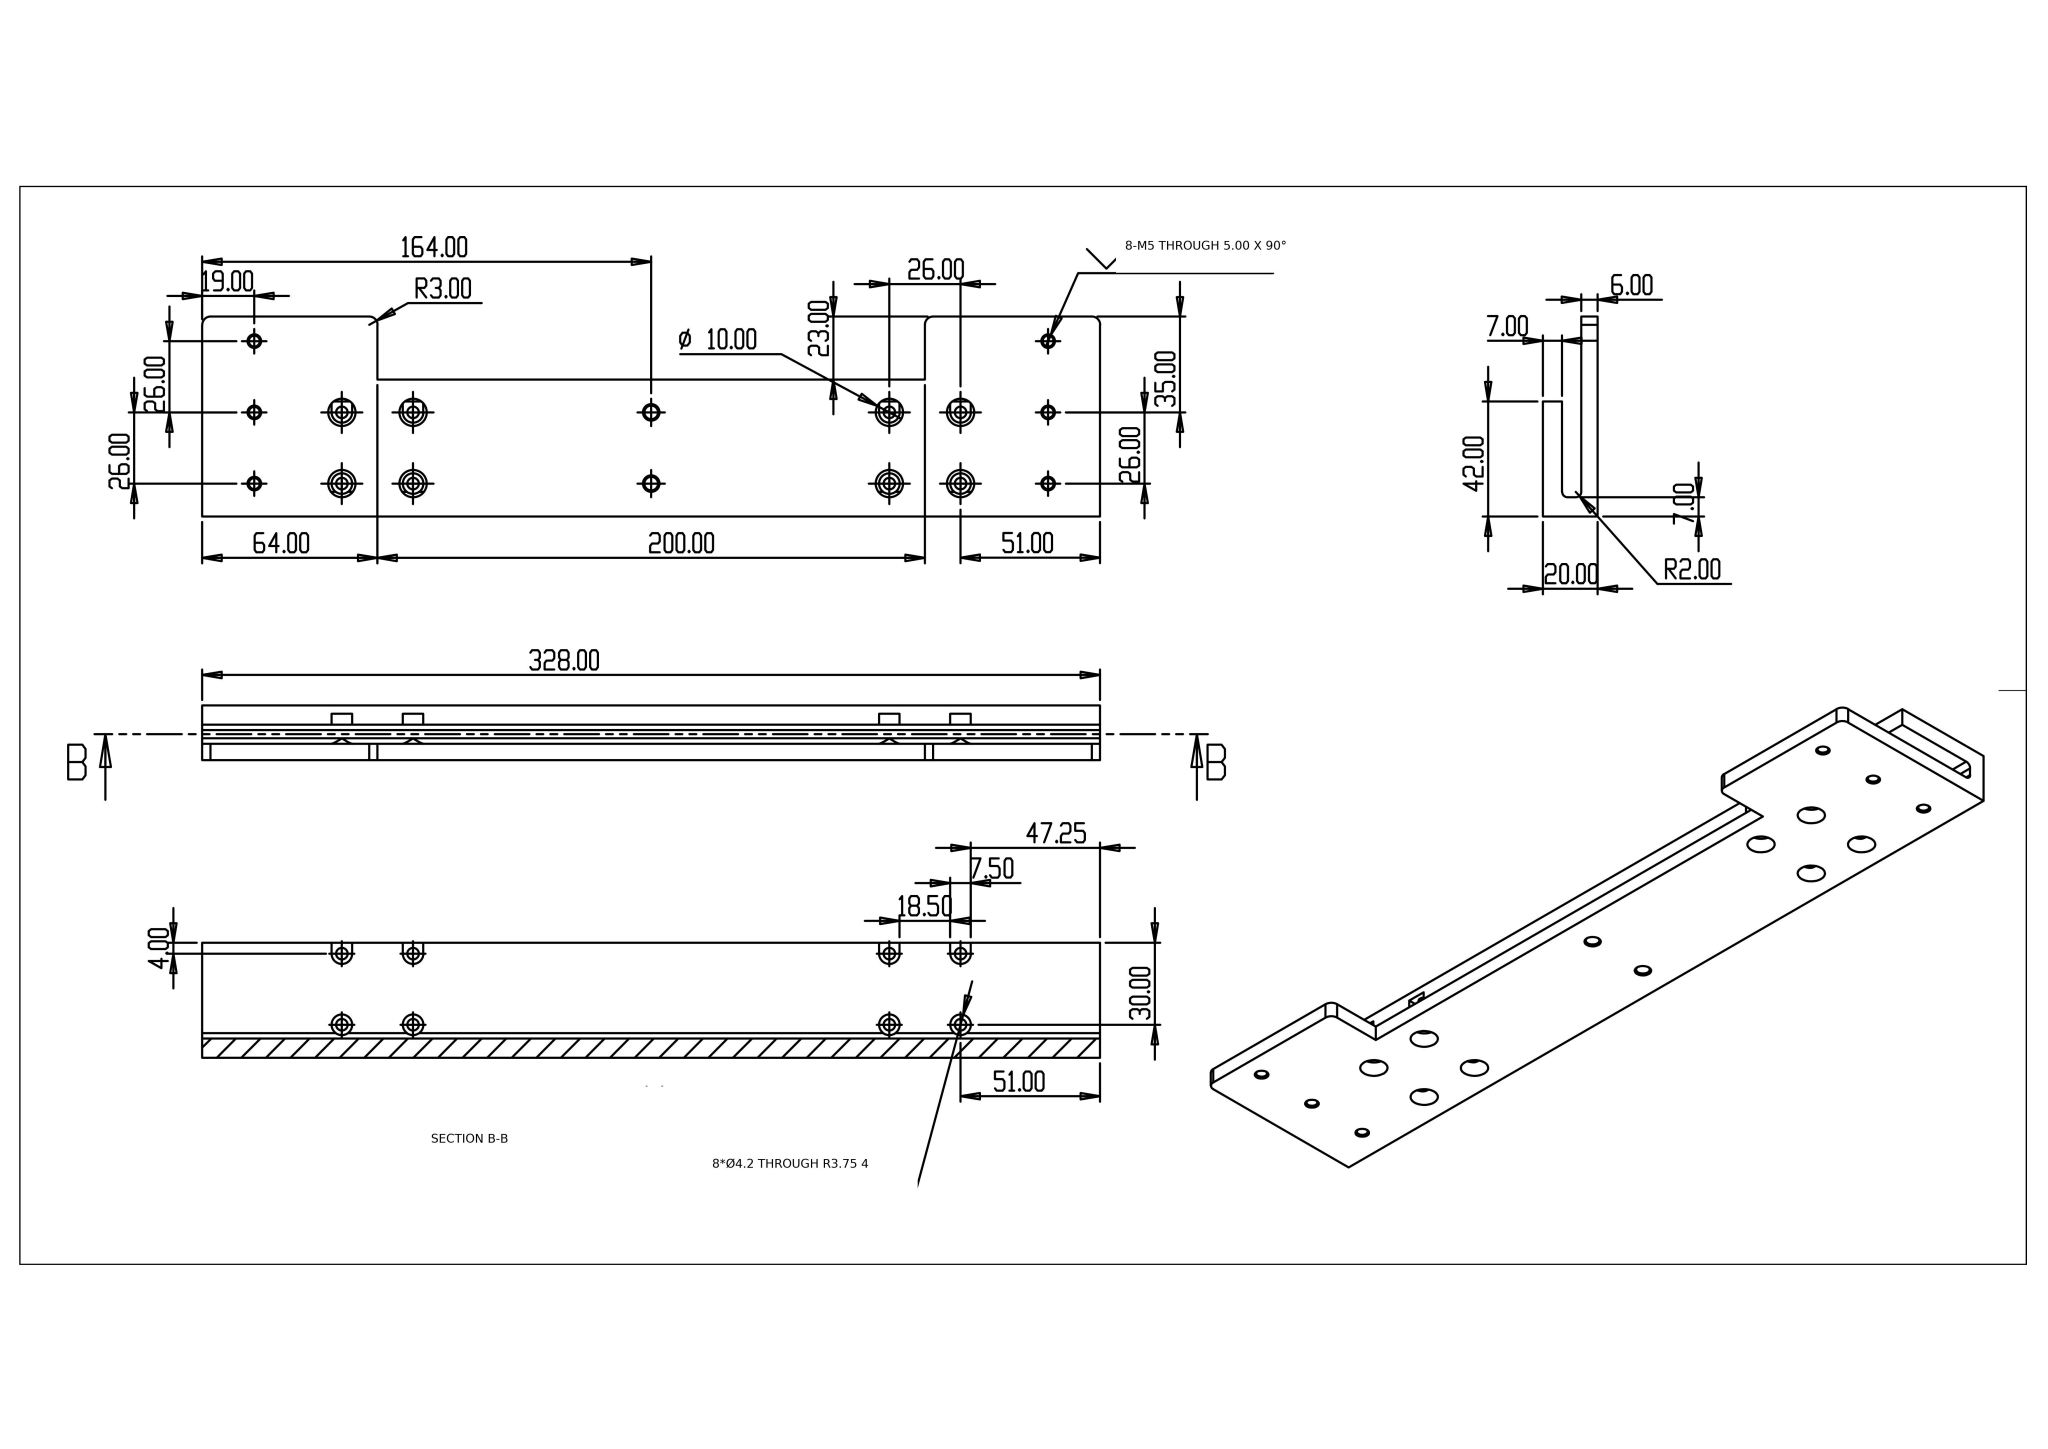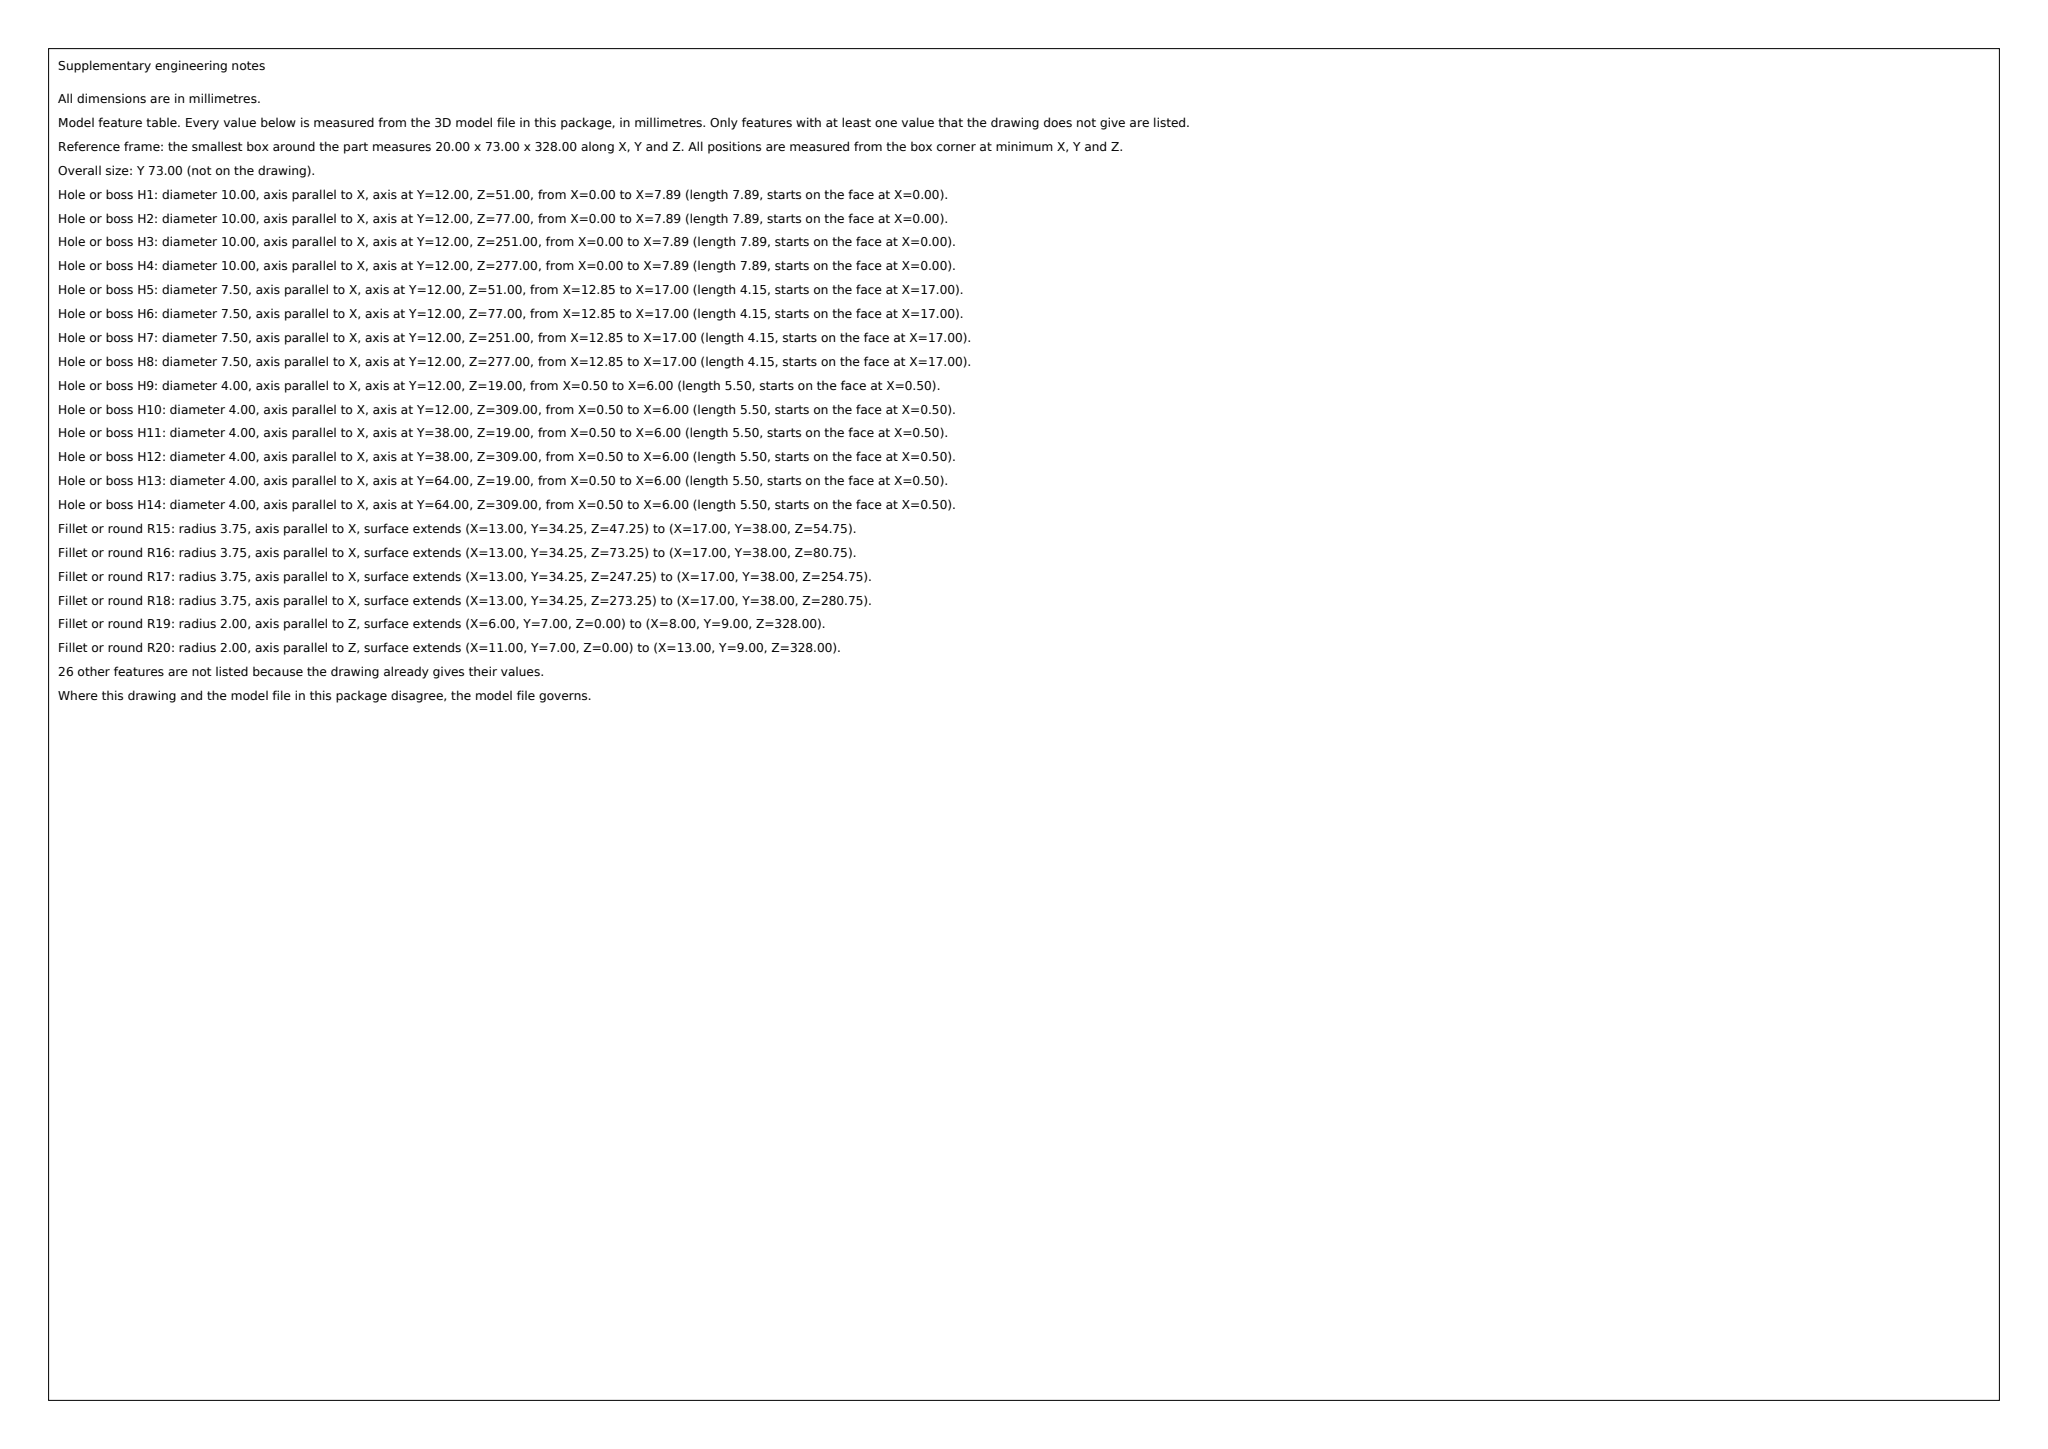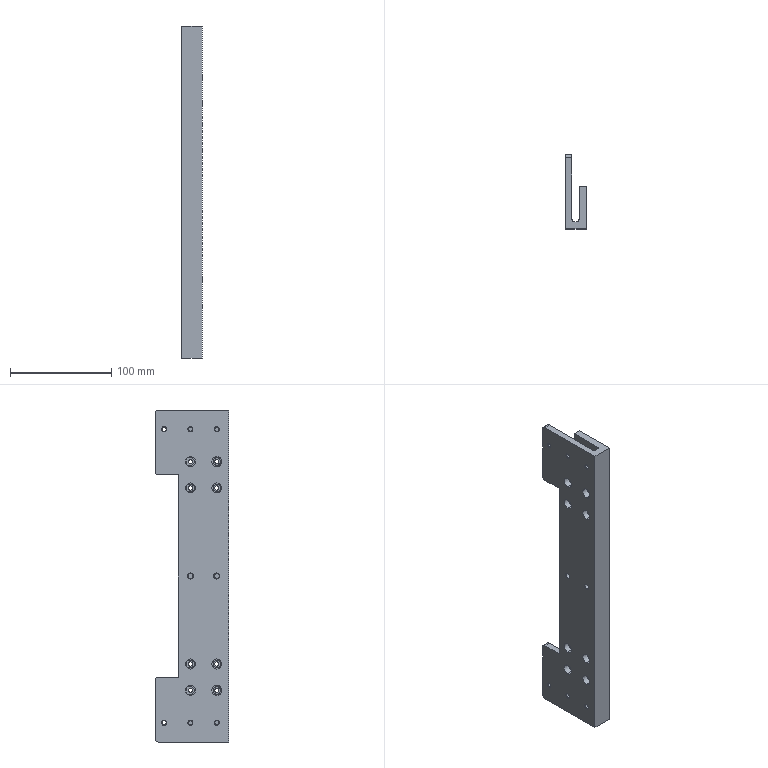Part | SolidWorks | mm | 1 solid | 112 faces | box 20 x 73 x 328 mm | volume 222727 mm3 | cylinder 66 | plane 30 | cone 16 | commonest cylinder face diameters 10 x16 4.2 x16 4 x14 7.5 x12 5 x4 6 x4
build123d program:
from build123d import *

# Parameters (mm, degrees)
BOSS_EXTRUDE1_DEPTH            = 328
CUT_EXTRUDE1_DEPTH             = 332.282
CUT_EXTRUDE2_REACH             = 333.282
SKETCH3_R                      = 2
CHAMFER1_SIZE                  = 0.5
SKETCH4_R                      = 3.75
SKETCH4_R_2                    = 3.75
CUT_EXTRUDE3_DEPTH             = 4
CUT_EXTRUDE3_DIRECTION_2_REACH = 332.934


with BuildPart() as part:
    # Sketch1 → Boss-Extrude1 (new body)
    with BuildSketch(Plane.XY):
        with BuildLine():
            Line((-20, 28), (-20, -42))
            Line((-20, -42), (0, -42))
            Line((0, -42), (0, 0))
            Line((0, 0), (-7, 0))
            Line((-7, 0), (-7, -33))
            ThreePointArc((-7, -33), (-7.586, -34.414), (-9, -35))
            Line((-9, -35), (-12, -35))
            ThreePointArc((-12, -35), (-13.414, -34.414), (-14, -33))
            Line((-14, -33), (-14, 28))
            Line((-14, 28), (-14, 31))
            Line((-14, 31), (-20, 31))
            Line((-20, 31), (-20, 28))
        make_face()
    extrude(amount=BOSS_EXTRUDE1_DEPTH)

    # Sketch2 → Cut-Extrude1 (cut, through all)
    with BuildSketch(Plane(origin=(0, 0, 0), x_dir=(0, 0, -1), z_dir=(1, 0, 0))):
        with BuildLine():
            Line((-64, 28), (-64, 8))
            Line((-64, 8), (-264, 8))
            Line((-264, 8), (-264, 28))
            ThreePointArc((-264, 28), (-264.879, 30.121), (-267, 31))
            Line((-267, 31), (-61, 31))
            ThreePointArc((-61, 31), (-63.121, 30.121), (-64, 28))
        make_face()
        with BuildLine():
            Line((-328, 28), (-328, 31))
            Line((-328, 31), (-325, 31))
            ThreePointArc((-325, 31), (-327.121, 30.121), (-328, 28))
        make_face()
        with BuildLine():
            Line((-3, 31), (0, 31))
            Line((0, 31), (0, 28))
            ThreePointArc((0, 28), (-0.8787, 30.121), (-3, 31))
        make_face()
        with BuildLine():
            ThreePointArc((-307, 22), (-309, 24), (-311, 22))
            ThreePointArc((-311, 22), (-309, 20), (-307, 22))
        make_face()
        with BuildLine():
            ThreePointArc((-17, 22), (-19, 24), (-21, 22))
            ThreePointArc((-21, 22), (-19, 20), (-17, 22))
        make_face()
        with BuildLine():
            ThreePointArc((-53.1, -4), (-51, -6.1), (-48.9, -4))
            ThreePointArc((-48.9, -4), (-51, -1.9), (-53.1, -4))
        make_face()
        with BuildLine():
            ThreePointArc((-253.1, -30), (-251, -32.1), (-248.9, -30))
            ThreePointArc((-248.9, -30), (-251, -27.9), (-253.1, -30))
        make_face()
        with BuildLine():
            ThreePointArc((-279.1, -30), (-277, -32.1), (-274.9, -30))
            ThreePointArc((-274.9, -30), (-277, -27.9), (-279.1, -30))
        make_face()
        with BuildLine():
            ThreePointArc((-253.1, -4), (-251, -6.1), (-248.9, -4))
            ThreePointArc((-248.9, -4), (-251, -1.9), (-253.1, -4))
        make_face()
        with BuildLine():
            ThreePointArc((-279.1, -4), (-277, -6.1), (-274.9, -4))
            ThreePointArc((-274.9, -4), (-277, -1.9), (-279.1, -4))
        make_face()
        with BuildLine():
            ThreePointArc((-79.1, -30), (-77, -32.1), (-74.9, -30))
            ThreePointArc((-74.9, -30), (-77, -27.9), (-79.1, -30))
        make_face()
        with BuildLine():
            ThreePointArc((-53.1, -30), (-51, -32.1), (-48.9, -30))
            ThreePointArc((-48.9, -30), (-51, -27.9), (-53.1, -30))
        make_face()
        with BuildLine():
            ThreePointArc((-79.1, -4), (-77, -6.1), (-74.9, -4))
            ThreePointArc((-74.9, -4), (-77, -1.9), (-79.1, -4))
        make_face()
    extrude(amount=-CUT_EXTRUDE1_DEPTH, mode=Mode.SUBTRACT)

    # Sketch3 → Cut-Extrude2 (cut, up to next)
    with BuildSketch(Plane.ZY.offset(20), mode=Mode.PRIVATE) as cut_extrude2_sk1:
        with Locations((309, -3.997)):
            Circle(SKETCH3_R)
    cut_extrude2_tool1 = extrude(cut_extrude2_sk1.sketch, amount=-CUT_EXTRUDE2_REACH, mode=Mode.PRIVATE) & part.part
    # Sketch3 → Cut-Extrude2 (cut, up to next)
    with BuildSketch(Plane.ZY.offset(20), mode=Mode.PRIVATE) as cut_extrude2_sk2:
        with Locations((309, -29.997)):
            Circle(SKETCH3_R)
    cut_extrude2_tool2 = extrude(cut_extrude2_sk2.sketch, amount=-CUT_EXTRUDE2_REACH, mode=Mode.PRIVATE) & part.part
    # Sketch3 → Cut-Extrude2 (cut, up to next)
    with BuildSketch(Plane.ZY.offset(20), mode=Mode.PRIVATE) as cut_extrude2_sk3:
        with Locations((19, -3.997)):
            Circle(SKETCH3_R)
    cut_extrude2_tool3 = extrude(cut_extrude2_sk3.sketch, amount=-CUT_EXTRUDE2_REACH, mode=Mode.PRIVATE) & part.part
    # Sketch3 → Cut-Extrude2 (cut, up to next)
    with BuildSketch(Plane.ZY.offset(20), mode=Mode.PRIVATE) as cut_extrude2_sk4:
        with Locations((19, -29.997)):
            Circle(SKETCH3_R)
    cut_extrude2_tool4 = extrude(cut_extrude2_sk4.sketch, amount=-CUT_EXTRUDE2_REACH, mode=Mode.PRIVATE) & part.part
    # Sketch3 → Cut-Extrude2 (cut, up to next)
    with BuildSketch(Plane.ZY.offset(20), mode=Mode.PRIVATE) as cut_extrude2_sk5:
        with BuildLine():
            ThreePointArc((282, -29.997), (277, -24.997), (272, -29.997))
            ThreePointArc((272, -29.997), (277, -34.997), (282, -29.997))
        make_face()
    cut_extrude2_tool5 = extrude(cut_extrude2_sk5.sketch, amount=-CUT_EXTRUDE2_REACH, mode=Mode.PRIVATE) & part.part
    # Sketch3 → Cut-Extrude2 (cut, up to next)
    with BuildSketch(Plane.ZY.offset(20), mode=Mode.PRIVATE) as cut_extrude2_sk6:
        with BuildLine():
            ThreePointArc((164, -27.497), (161.5, -29.997), (164, -32.497))
            ThreePointArc((164, -32.497), (166.5, -29.997), (164, -27.497))
        make_face()
    cut_extrude2_tool6 = extrude(cut_extrude2_sk6.sketch, amount=-CUT_EXTRUDE2_REACH, mode=Mode.PRIVATE) & part.part
    # Sketch3 → Cut-Extrude2 (cut, up to next)
    with BuildSketch(Plane.ZY.offset(20), mode=Mode.PRIVATE) as cut_extrude2_sk7:
        with BuildLine():
            ThreePointArc((164, -1.497), (161.5, -3.997), (164, -6.497))
            ThreePointArc((164, -6.497), (166.5, -3.997), (164, -1.497))
        make_face()
    cut_extrude2_tool7 = extrude(cut_extrude2_sk7.sketch, amount=-CUT_EXTRUDE2_REACH, mode=Mode.PRIVATE) & part.part
    # Sketch3 → Cut-Extrude2 (cut, up to next)
    with BuildSketch(Plane.ZY.offset(20), mode=Mode.PRIVATE) as cut_extrude2_sk8:
        with BuildLine():
            ThreePointArc((56, -3.997), (51, 1.003), (46, -3.997))
            ThreePointArc((46, -3.997), (51, -8.997), (56, -3.997))
        make_face()
    cut_extrude2_tool8 = extrude(cut_extrude2_sk8.sketch, amount=-CUT_EXTRUDE2_REACH, mode=Mode.PRIVATE) & part.part
    # Sketch3 → Cut-Extrude2 (cut, up to next)
    with BuildSketch(Plane.ZY.offset(20), mode=Mode.PRIVATE) as cut_extrude2_sk9:
        with BuildLine():
            ThreePointArc((82, -29.997), (77, -24.997), (72, -29.997))
            ThreePointArc((72, -29.997), (77, -34.997), (82, -29.997))
        make_face()
    cut_extrude2_tool9 = extrude(cut_extrude2_sk9.sketch, amount=-CUT_EXTRUDE2_REACH, mode=Mode.PRIVATE) & part.part
    # Sketch3 → Cut-Extrude2 (cut, up to next)
    with BuildSketch(Plane.ZY.offset(20), mode=Mode.PRIVATE) as cut_extrude2_sk10:
        with BuildLine():
            ThreePointArc((256, -29.997), (251, -24.997), (246, -29.997))
            ThreePointArc((246, -29.997), (251, -34.997), (256, -29.997))
        make_face()
    cut_extrude2_tool10 = extrude(cut_extrude2_sk10.sketch, amount=-CUT_EXTRUDE2_REACH, mode=Mode.PRIVATE) & part.part
    # Sketch3 → Cut-Extrude2 (cut, up to next)
    with BuildSketch(Plane.ZY.offset(20), mode=Mode.PRIVATE) as cut_extrude2_sk11:
        with BuildLine():
            ThreePointArc((256, -3.997), (251, 1.003), (246, -3.997))
            ThreePointArc((246, -3.997), (251, -8.997), (256, -3.997))
        make_face()
    cut_extrude2_tool11 = extrude(cut_extrude2_sk11.sketch, amount=-CUT_EXTRUDE2_REACH, mode=Mode.PRIVATE) & part.part
    # Sketch3 → Cut-Extrude2 (cut, up to next)
    with BuildSketch(Plane.ZY.offset(20), mode=Mode.PRIVATE) as cut_extrude2_sk12:
        with BuildLine():
            ThreePointArc((82, -3.997), (77, 1.003), (72, -3.997))
            ThreePointArc((72, -3.997), (77, -8.997), (82, -3.997))
        make_face()
    cut_extrude2_tool12 = extrude(cut_extrude2_sk12.sketch, amount=-CUT_EXTRUDE2_REACH, mode=Mode.PRIVATE) & part.part
    # Sketch3 → Cut-Extrude2 (cut, up to next)
    with BuildSketch(Plane.ZY.offset(20), mode=Mode.PRIVATE) as cut_extrude2_sk13:
        with BuildLine():
            ThreePointArc((56, -29.997), (51, -24.997), (46, -29.997))
            ThreePointArc((46, -29.997), (51, -34.997), (56, -29.997))
        make_face()
    cut_extrude2_tool13 = extrude(cut_extrude2_sk13.sketch, amount=-CUT_EXTRUDE2_REACH, mode=Mode.PRIVATE) & part.part
    # Sketch3 → Cut-Extrude2 (cut, up to next)
    with BuildSketch(Plane.ZY.offset(20), mode=Mode.PRIVATE) as cut_extrude2_sk14:
        with BuildLine():
            ThreePointArc((282, -3.997), (277, 1.003), (272, -3.997))
            ThreePointArc((272, -3.997), (277, -8.997), (282, -3.997))
        make_face()
    cut_extrude2_tool14 = extrude(cut_extrude2_sk14.sketch, amount=-CUT_EXTRUDE2_REACH, mode=Mode.PRIVATE) & part.part
    add(cut_extrude2_tool1.solids().sort_by_distance((-20, -3.997, 309))[0], mode=Mode.SUBTRACT)
    add(cut_extrude2_tool2.solids().sort_by_distance((-20, -29.997, 309))[0], mode=Mode.SUBTRACT)
    add(cut_extrude2_tool3.solids().sort_by_distance((-20, -3.997, 19))[0], mode=Mode.SUBTRACT)
    add(cut_extrude2_tool4.solids().sort_by_distance((-20, -29.997, 19))[0], mode=Mode.SUBTRACT)
    add(cut_extrude2_tool5.solids().sort_by_distance((-20, -29.997, 277))[0], mode=Mode.SUBTRACT)
    add(cut_extrude2_tool6.solids().sort_by_distance((-20, -29.997, 164))[0], mode=Mode.SUBTRACT)
    add(cut_extrude2_tool7.solids().sort_by_distance((-20, -3.997, 164))[0], mode=Mode.SUBTRACT)
    add(cut_extrude2_tool8.solids().sort_by_distance((-20, -3.997, 51))[0], mode=Mode.SUBTRACT)
    add(cut_extrude2_tool9.solids().sort_by_distance((-20, -29.997, 77))[0], mode=Mode.SUBTRACT)
    add(cut_extrude2_tool10.solids().sort_by_distance((-20, -29.997, 251))[0], mode=Mode.SUBTRACT)
    add(cut_extrude2_tool11.solids().sort_by_distance((-20, -3.997, 251))[0], mode=Mode.SUBTRACT)
    add(cut_extrude2_tool12.solids().sort_by_distance((-20, -3.997, 77))[0], mode=Mode.SUBTRACT)
    add(cut_extrude2_tool13.solids().sort_by_distance((-20, -29.997, 51))[0], mode=Mode.SUBTRACT)
    add(cut_extrude2_tool14.solids().sort_by_distance((-20, -3.997, 277))[0], mode=Mode.SUBTRACT)

    # Chamfer1
    chamfer1_edges = [part.edges().sort_by_distance(p)[0] for p in [
        (-20, 22, 311),
        (-20, 22, 17),
        (-20, -6.497, 164),
        (-20, -32.497, 164),
        (-20, -29.997, 17),
        (-20, -3.997, 17),
        (-20, -29.997, 307),
        (-20, -3.997, 307),
    ]]
    chamfer(chamfer1_edges, length=CHAMFER1_SIZE)

    # Sketch4 → Cut-Extrude3 (cut)
    with BuildSketch(Plane.ZY.offset(7)):
        with Locations(Location((51, -30, 0), (0, 0, 233.13))):
            Circle(SKETCH4_R)
        with Locations(Location((77, -30, 0), (0, 0, 233.13))):
            Circle(SKETCH4_R)
        with Locations(Location((251, -30, 0), (0, 0, 233.13))):
            Circle(SKETCH4_R)
        with Locations(Location((277, -30, 0), (0, 0, 233.13))):
            Circle(SKETCH4_R_2)
        with BuildLine():
            Line((47.25, -4), (47.25, 0))
            Line((47.25, 0), (54.75, 0))
            Line((54.75, 0), (54.75, -4))
            ThreePointArc((54.75, -4), (51, -7.75), (47.25, -4))
        make_face()
        with BuildLine():
            Line((280.75, 0), (280.75, -4))
            ThreePointArc((280.75, -4), (277, -7.75), (273.25, -4))
            Line((273.25, -4), (273.25, 0))
            Line((273.25, 0), (280.75, 0))
        make_face()
        with BuildLine():
            Line((254.75, 0), (254.75, -4))
            ThreePointArc((254.75, -4), (251, -7.75), (247.25, -4))
            Line((247.25, -4), (247.25, 0))
            Line((247.25, 0), (254.75, 0))
        make_face()
        with BuildLine():
            Line((80.75, 0), (80.75, -4))
            ThreePointArc((80.75, -4), (77, -7.75), (73.25, -4))
            Line((73.25, -4), (73.25, 0))
            Line((73.25, 0), (80.75, 0))
        make_face()
    extrude(amount=-CUT_EXTRUDE3_DEPTH, mode=Mode.SUBTRACT)

    # Cut-Extrude3 direction 2: up to this face of the body (flat: up to its plane)
    cut_extrude3_direction_2_end = Plane(part.part.faces().sort_by_distance((-14, -2.5, 3.342))[0])
    # Sketch4 → Cut-Extrude3 direction 2 (cut, up to the picked face)
    with BuildSketch(Plane.ZY.offset(7), mode=Mode.PRIVATE) as cut_extrude3_direction_2_sk1:
        with Locations(Location((51, -30, 0), (0, 0, 233.13))):
            Circle(SKETCH4_R)
    cut_extrude3_direction_2_tool1 = split(extrude(cut_extrude3_direction_2_sk1.sketch, amount=CUT_EXTRUDE3_DIRECTION_2_REACH, mode=Mode.PRIVATE), bisect_by=cut_extrude3_direction_2_end, keep=Keep.BOTH, mode=Mode.PRIVATE)
    # Sketch4 → Cut-Extrude3 direction 2 (cut, up to the picked face)
    with BuildSketch(Plane.ZY.offset(7), mode=Mode.PRIVATE) as cut_extrude3_direction_2_sk2:
        with Locations(Location((77, -30, 0), (0, 0, 233.13))):
            Circle(SKETCH4_R)
    cut_extrude3_direction_2_tool2 = split(extrude(cut_extrude3_direction_2_sk2.sketch, amount=CUT_EXTRUDE3_DIRECTION_2_REACH, mode=Mode.PRIVATE), bisect_by=cut_extrude3_direction_2_end, keep=Keep.BOTH, mode=Mode.PRIVATE)
    # Sketch4 → Cut-Extrude3 direction 2 (cut, up to the picked face)
    with BuildSketch(Plane.ZY.offset(7), mode=Mode.PRIVATE) as cut_extrude3_direction_2_sk3:
        with Locations(Location((251, -30, 0), (0, 0, 233.13))):
            Circle(SKETCH4_R)
    cut_extrude3_direction_2_tool3 = split(extrude(cut_extrude3_direction_2_sk3.sketch, amount=CUT_EXTRUDE3_DIRECTION_2_REACH, mode=Mode.PRIVATE), bisect_by=cut_extrude3_direction_2_end, keep=Keep.BOTH, mode=Mode.PRIVATE)
    # Sketch4 → Cut-Extrude3 direction 2 (cut, up to the picked face)
    with BuildSketch(Plane.ZY.offset(7), mode=Mode.PRIVATE) as cut_extrude3_direction_2_sk4:
        with Locations(Location((277, -30, 0), (0, 0, 233.13))):
            Circle(SKETCH4_R_2)
    cut_extrude3_direction_2_tool4 = split(extrude(cut_extrude3_direction_2_sk4.sketch, amount=CUT_EXTRUDE3_DIRECTION_2_REACH, mode=Mode.PRIVATE), bisect_by=cut_extrude3_direction_2_end, keep=Keep.BOTH, mode=Mode.PRIVATE)
    # Sketch4 → Cut-Extrude3 direction 2 (cut, up to the picked face)
    with BuildSketch(Plane.ZY.offset(7), mode=Mode.PRIVATE) as cut_extrude3_direction_2_sk5:
        with BuildLine():
            Line((47.25, -4), (47.25, 0))
            Line((47.25, 0), (54.75, 0))
            Line((54.75, 0), (54.75, -4))
            ThreePointArc((54.75, -4), (51, -7.75), (47.25, -4))
        make_face()
    cut_extrude3_direction_2_tool5 = split(extrude(cut_extrude3_direction_2_sk5.sketch, amount=CUT_EXTRUDE3_DIRECTION_2_REACH, mode=Mode.PRIVATE), bisect_by=cut_extrude3_direction_2_end, keep=Keep.BOTH, mode=Mode.PRIVATE)
    # Sketch4 → Cut-Extrude3 direction 2 (cut, up to the picked face)
    with BuildSketch(Plane.ZY.offset(7), mode=Mode.PRIVATE) as cut_extrude3_direction_2_sk6:
        with BuildLine():
            Line((280.75, 0), (280.75, -4))
            ThreePointArc((280.75, -4), (277, -7.75), (273.25, -4))
            Line((273.25, -4), (273.25, 0))
            Line((273.25, 0), (280.75, 0))
        make_face()
    cut_extrude3_direction_2_tool6 = split(extrude(cut_extrude3_direction_2_sk6.sketch, amount=CUT_EXTRUDE3_DIRECTION_2_REACH, mode=Mode.PRIVATE), bisect_by=cut_extrude3_direction_2_end, keep=Keep.BOTH, mode=Mode.PRIVATE)
    # Sketch4 → Cut-Extrude3 direction 2 (cut, up to the picked face)
    with BuildSketch(Plane.ZY.offset(7), mode=Mode.PRIVATE) as cut_extrude3_direction_2_sk7:
        with BuildLine():
            Line((254.75, 0), (254.75, -4))
            ThreePointArc((254.75, -4), (251, -7.75), (247.25, -4))
            Line((247.25, -4), (247.25, 0))
            Line((247.25, 0), (254.75, 0))
        make_face()
    cut_extrude3_direction_2_tool7 = split(extrude(cut_extrude3_direction_2_sk7.sketch, amount=CUT_EXTRUDE3_DIRECTION_2_REACH, mode=Mode.PRIVATE), bisect_by=cut_extrude3_direction_2_end, keep=Keep.BOTH, mode=Mode.PRIVATE)
    # Sketch4 → Cut-Extrude3 direction 2 (cut, up to the picked face)
    with BuildSketch(Plane.ZY.offset(7), mode=Mode.PRIVATE) as cut_extrude3_direction_2_sk8:
        with BuildLine():
            Line((80.75, 0), (80.75, -4))
            ThreePointArc((80.75, -4), (77, -7.75), (73.25, -4))
            Line((73.25, -4), (73.25, 0))
            Line((73.25, 0), (80.75, 0))
        make_face()
    cut_extrude3_direction_2_tool8 = split(extrude(cut_extrude3_direction_2_sk8.sketch, amount=CUT_EXTRUDE3_DIRECTION_2_REACH, mode=Mode.PRIVATE), bisect_by=cut_extrude3_direction_2_end, keep=Keep.BOTH, mode=Mode.PRIVATE)
    add(cut_extrude3_direction_2_tool1.solids().sort_by(Axis((-7, -30, 51), (-1, 0, 0)))[0], mode=Mode.SUBTRACT)
    add(cut_extrude3_direction_2_tool2.solids().sort_by(Axis((-7, -30, 77), (-1, 0, 0)))[0], mode=Mode.SUBTRACT)
    add(cut_extrude3_direction_2_tool3.solids().sort_by(Axis((-7, -30, 251), (-1, 0, 0)))[0], mode=Mode.SUBTRACT)
    add(cut_extrude3_direction_2_tool4.solids().sort_by(Axis((-7, -30, 277), (-1, 0, 0)))[0], mode=Mode.SUBTRACT)
    add(cut_extrude3_direction_2_tool5.solids().sort_by(Axis((-7, -3.523, 51), (-1, 0, 0)))[0], mode=Mode.SUBTRACT)
    add(cut_extrude3_direction_2_tool6.solids().sort_by(Axis((-7, -3.523, 277), (-1, 0, 0)))[0], mode=Mode.SUBTRACT)
    add(cut_extrude3_direction_2_tool7.solids().sort_by(Axis((-7, -3.523, 251), (-1, 0, 0)))[0], mode=Mode.SUBTRACT)
    add(cut_extrude3_direction_2_tool8.solids().sort_by(Axis((-7, -3.523, 77), (-1, 0, 0)))[0], mode=Mode.SUBTRACT)


solid = part.part